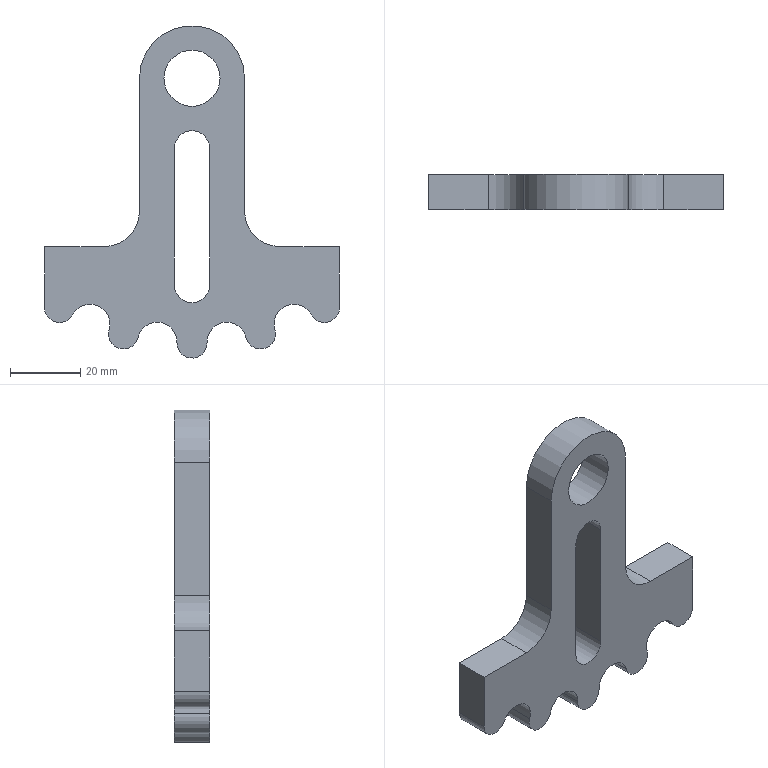Component | NX | 6_BALANCE_WHEEL | 1 solid | 25 faces | volume 31016 mm3 | cylinder 15 | plane 10 | commonest cylinder face diameters 8.6 x5 11.2 x4 10 x2 20 x2 30 x1 16 x1